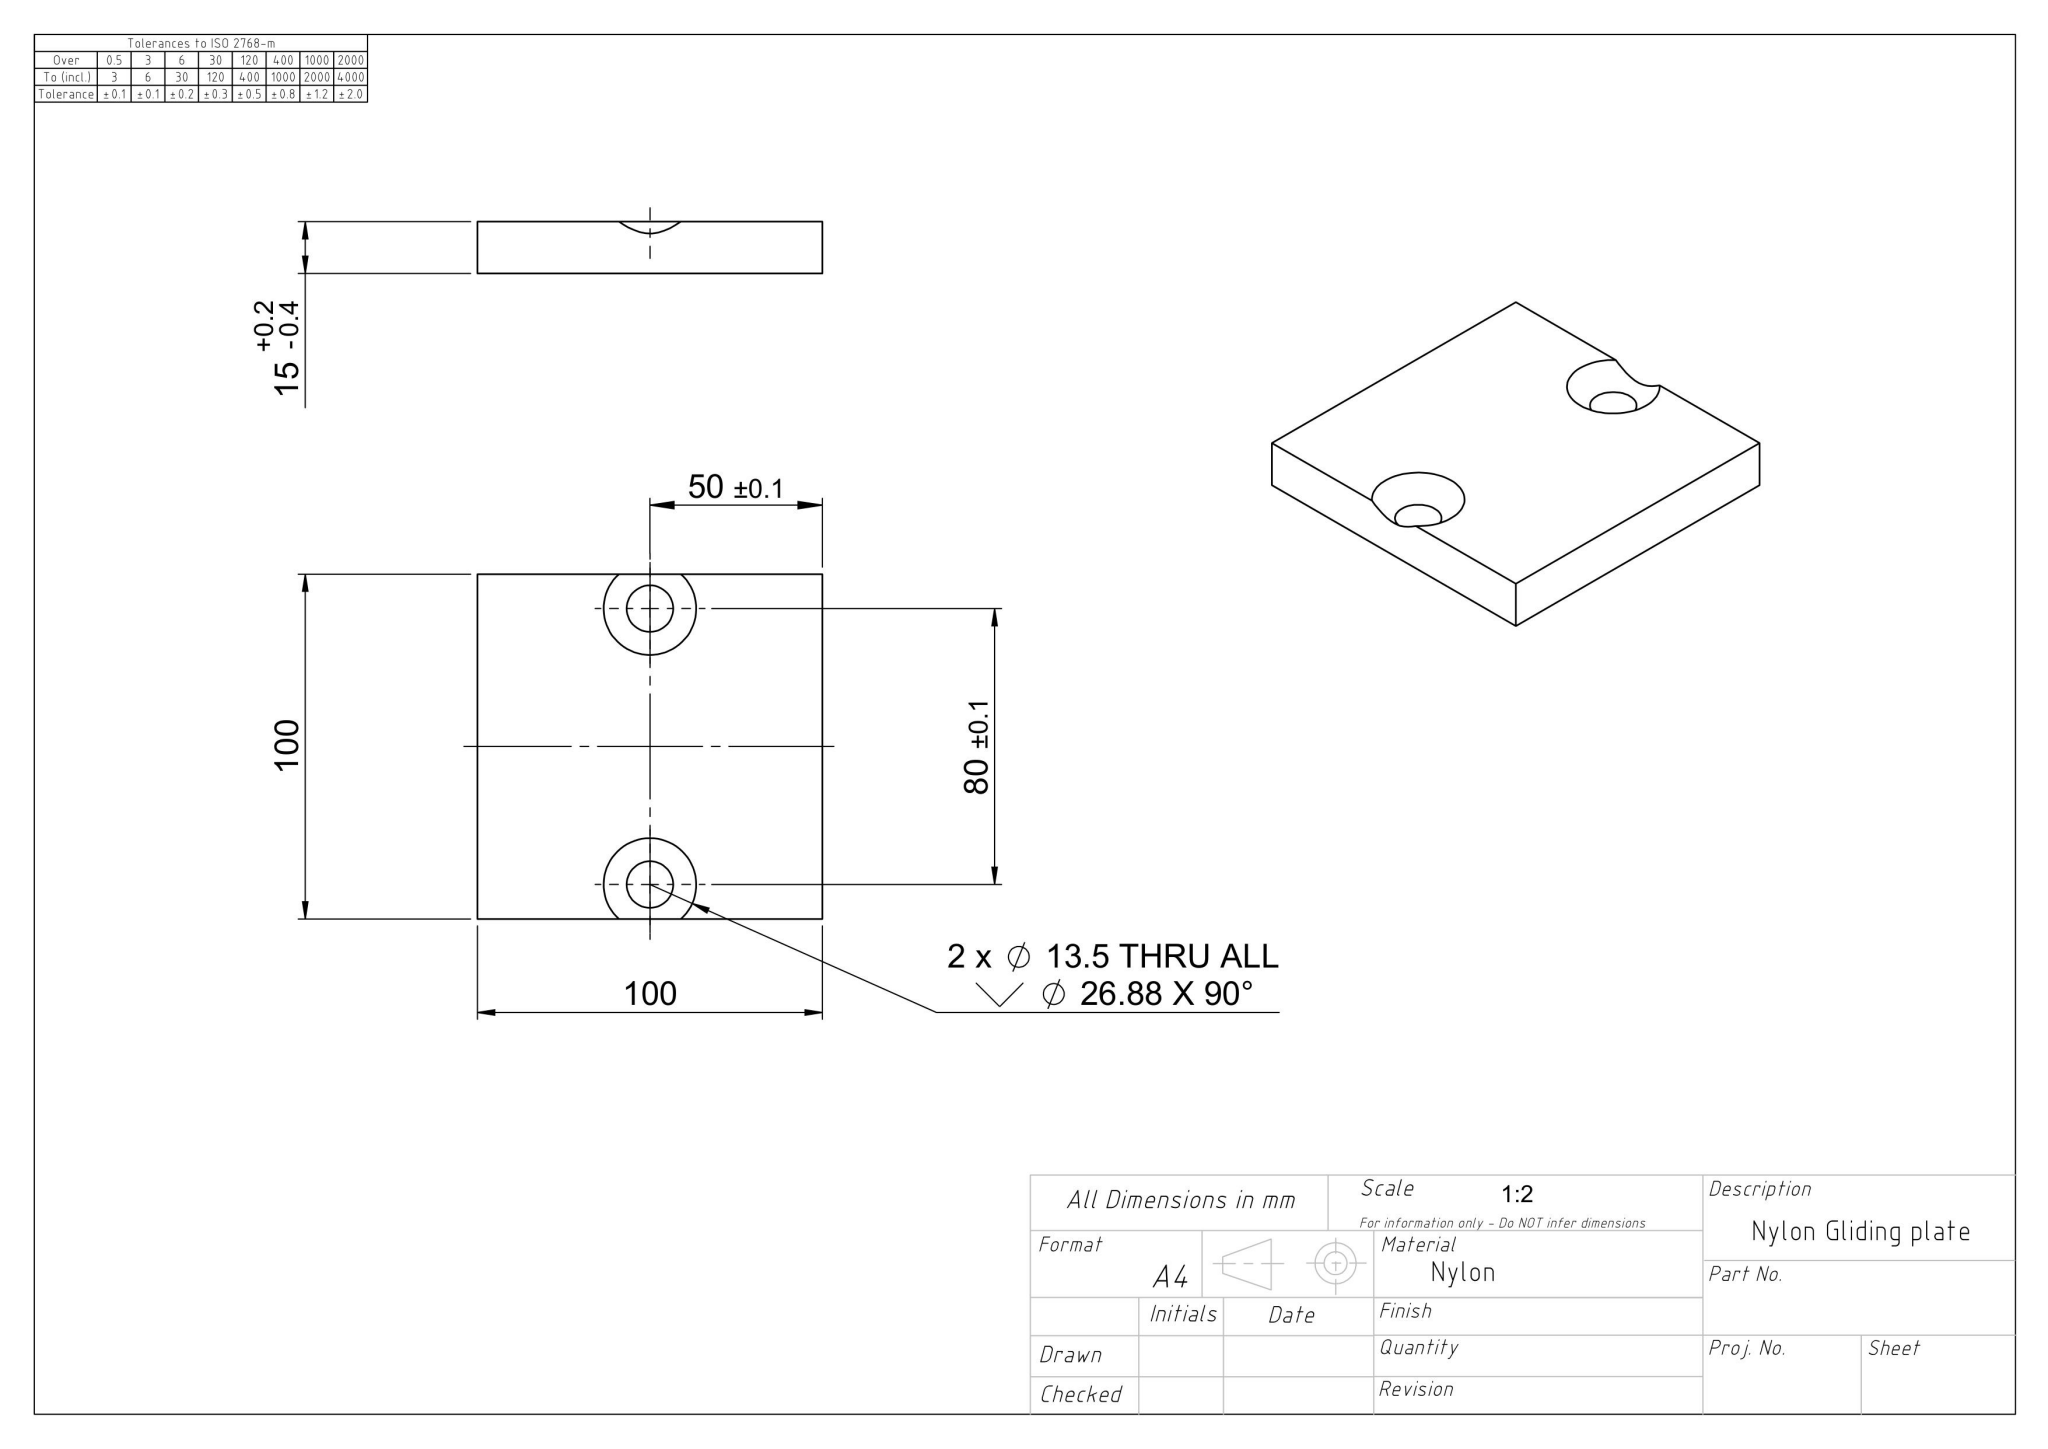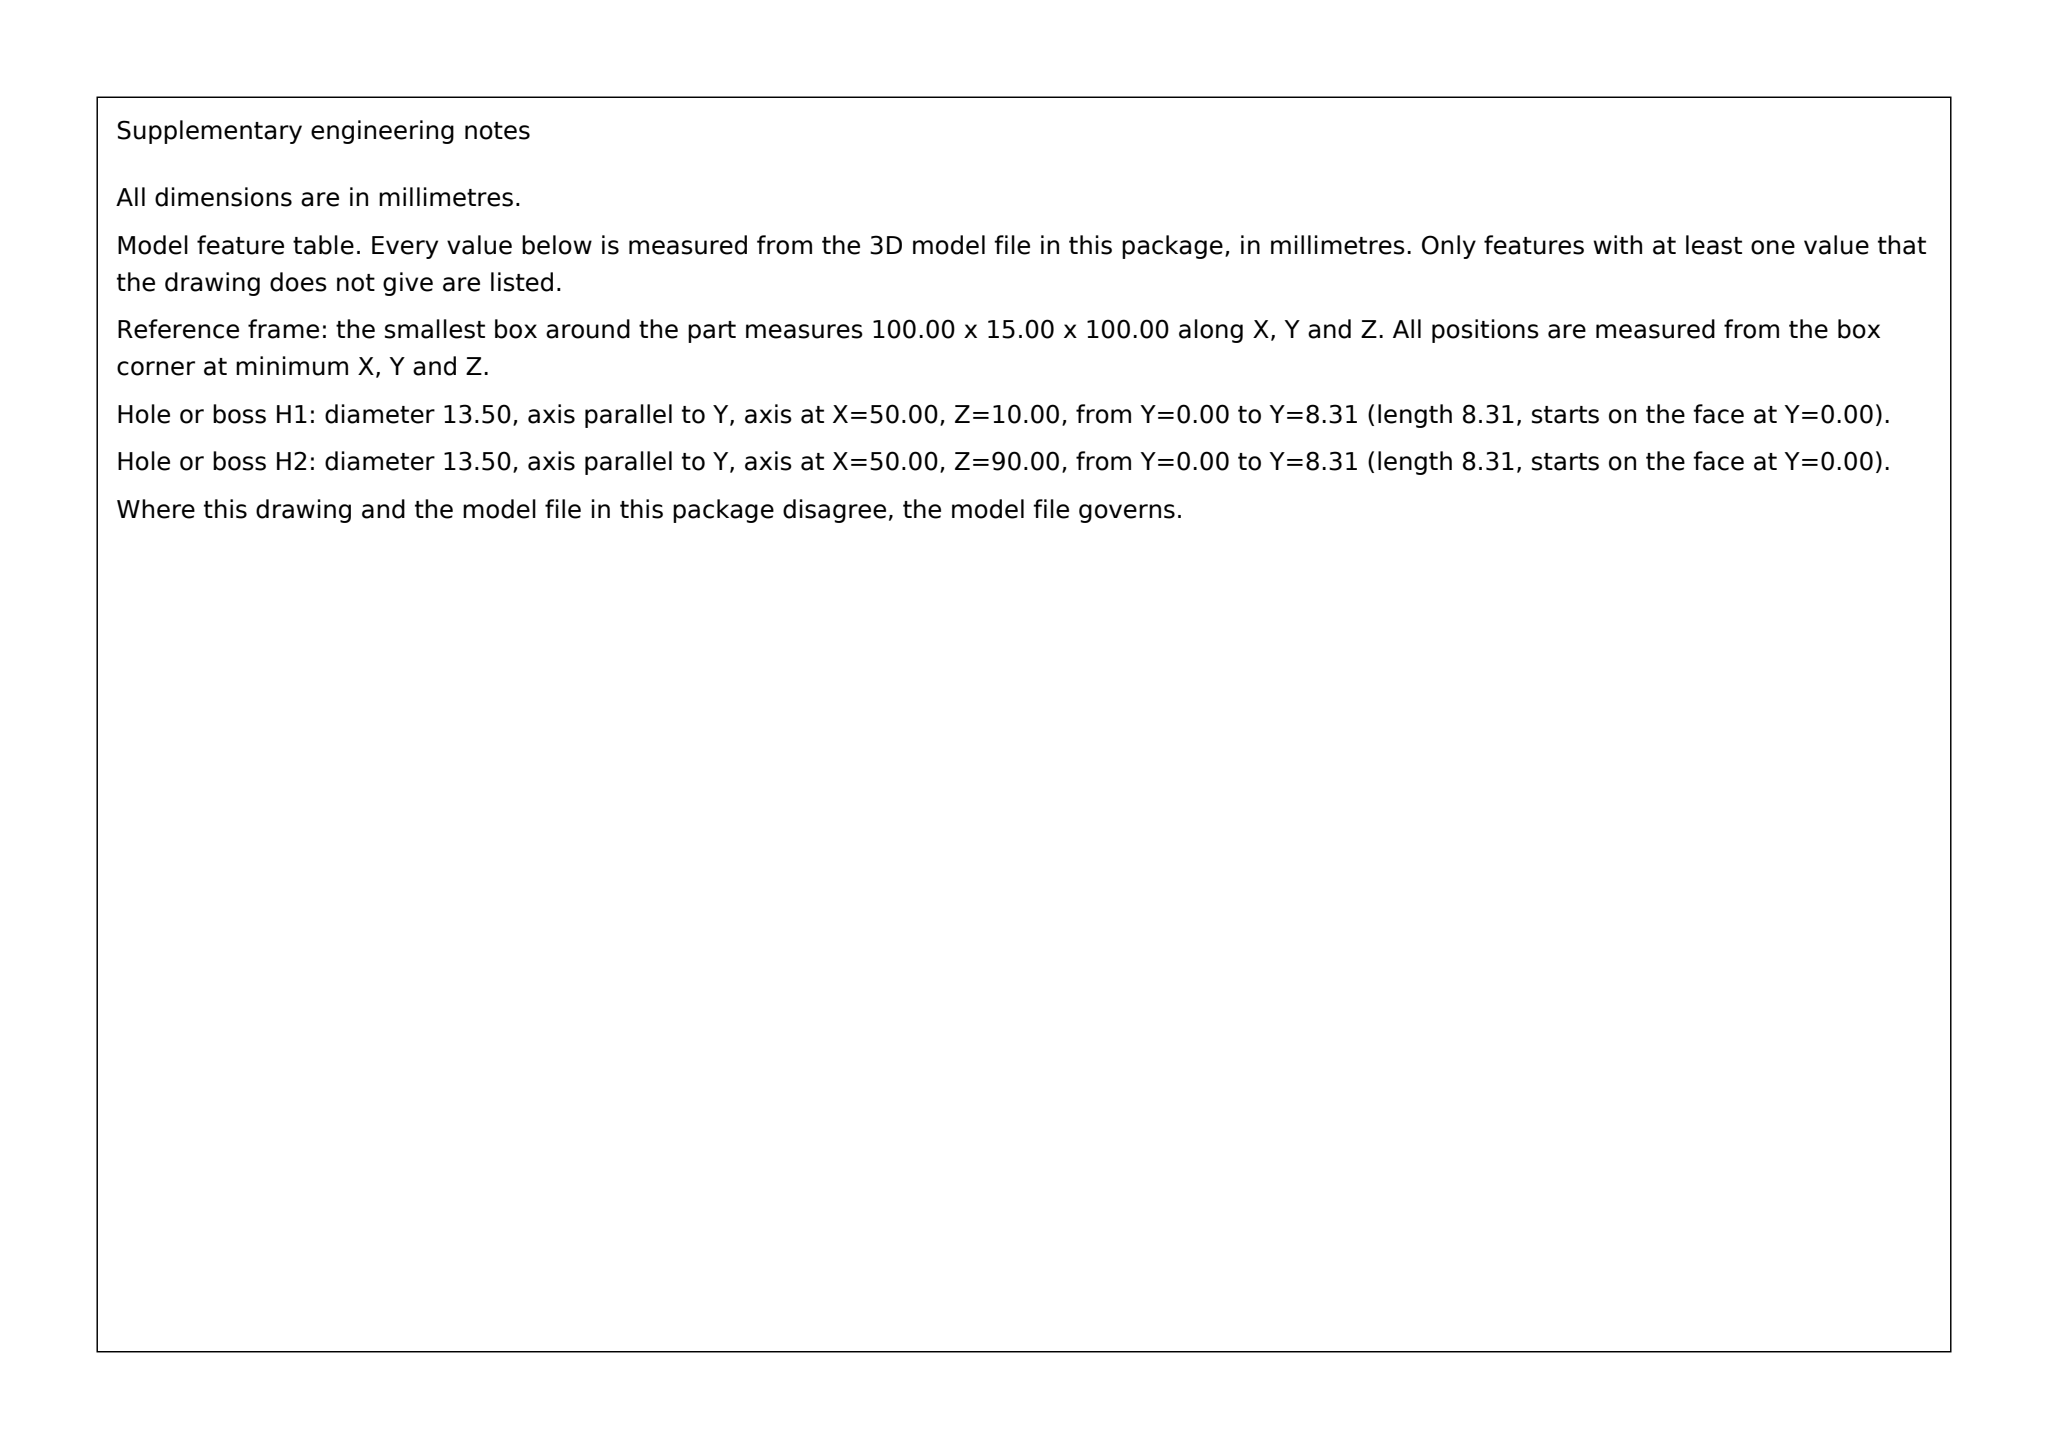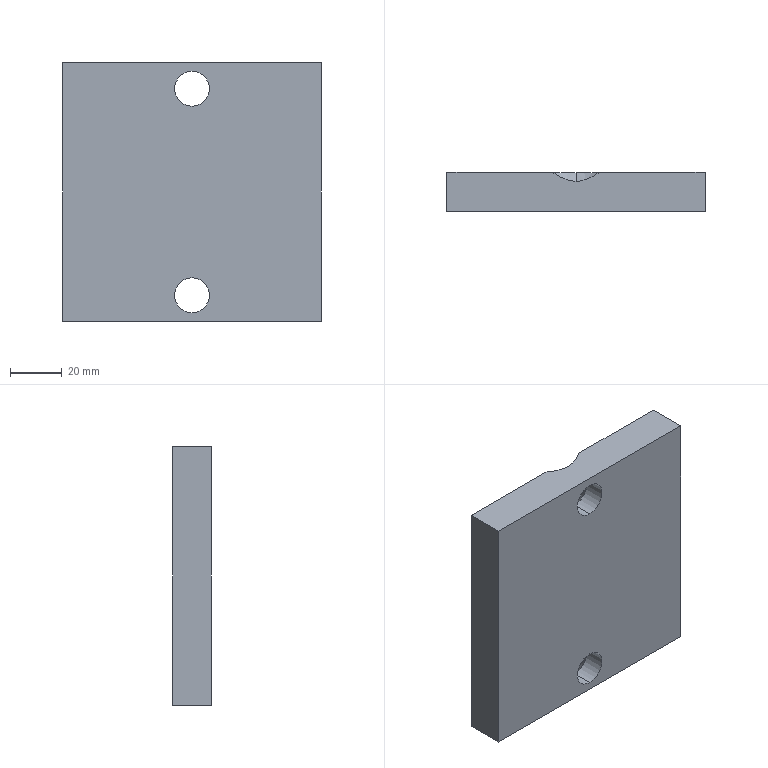Part | SolidWorks | mm | material Nylon | 1 solid | 14 faces | box 100 x 15 x 100 mm | volume 143294 mm3 | plane 6 | cylinder 4 | cone 4 | commonest cylinder face diameters 13.5 x4
build123d program:
from build123d import *

# Parameters (mm, degrees)
SKETCH4_W                                            = 100
SKETCH4_H                                            = 100
BOSS_EXTRUDE3_DEPTH                                  = 15
CSK_FOR_M12_HEX_SOCKET_COUNTERSUNK_CAP_S_D           = 13.5
CSK_FOR_M12_HEX_SOCKET_COUNTERSUNK_CAP_S_CSINK_D     = 26.88
CSK_FOR_M12_HEX_SOCKET_COUNTERSUNK_CAP_S_CSINK_ANGLE = 90


with BuildPart() as part:
    # Sketch4 → Boss-Extrude3 (new body)
    with BuildSketch(Plane(origin=(0, 0, 0), x_dir=(1, 0, 0), z_dir=(0, 1, 0))):
        Rectangle(SKETCH4_W, SKETCH4_H)
    extrude(amount=BOSS_EXTRUDE3_DEPTH)

    # CSK for M12 Hex Socket Countersunk Cap S (through all)
    with Locations(Plane(origin=(0, 15, 0), x_dir=(1, 0, 0), z_dir=(0, 1, 0))):
        with Locations((0, 40), (0, -40)):
            CounterSinkHole(CSK_FOR_M12_HEX_SOCKET_COUNTERSUNK_CAP_S_D / 2, CSK_FOR_M12_HEX_SOCKET_COUNTERSUNK_CAP_S_CSINK_D / 2, counter_sink_angle=CSK_FOR_M12_HEX_SOCKET_COUNTERSUNK_CAP_S_CSINK_ANGLE)


solid = part.part
STEP:
#1=CARTESIAN_POINT('',(0.,0.,-46.75));
#2=VERTEX_POINT('',#1);
#3=CARTESIAN_POINT('',(0.,0.,-33.25));
#4=VERTEX_POINT('',#3);
#5=CARTESIAN_POINT('',(0.,0.,-40.));
#6=DIRECTION('',(0.,1.,0.));
#7=DIRECTION('',(0.,0.,1.));
#8=AXIS2_PLACEMENT_3D('',#5,#6,#7);
#9=CIRCLE('',#8,6.75);
#10=EDGE_CURVE('',#2,#4,#9,.T.);
#11=ORIENTED_EDGE('',*,*,#10,.F.);
#12=CARTESIAN_POINT('',(0.,8.31,-46.75));
#13=VERTEX_POINT('',#12);
#14=CARTESIAN_POINT('',(0.,15.,-46.75));
#15=DIRECTION('',(0.,1.,0.));
#16=VECTOR('',#15,1000.);
#17=LINE('',#14,#16);
#18=EDGE_CURVE('',#2,#13,#17,.T.);
#19=ORIENTED_EDGE('',*,*,#18,.T.);
#20=CARTESIAN_POINT('',(0.,8.31,-33.25));
#21=VERTEX_POINT('',#20);
#22=CARTESIAN_POINT('',(0.,8.31,-40.));
#23=DIRECTION('',(0.,1.,0.));
#24=DIRECTION('',(0.,0.,1.));
#25=AXIS2_PLACEMENT_3D('',#22,#23,#24);
#26=CIRCLE('',#25,6.75);
#27=EDGE_CURVE('',#13,#21,#26,.T.);
#28=ORIENTED_EDGE('',*,*,#27,.T.);
#29=CARTESIAN_POINT('',(0.,15.,-33.25));
#30=DIRECTION('',(0.,1.,0.));
#31=VECTOR('',#30,1000.);
#32=LINE('',#29,#31);
#33=EDGE_CURVE('',#4,#21,#32,.T.);
#34=ORIENTED_EDGE('',*,*,#33,.F.);
#35=EDGE_LOOP('',(#11,#19,#28,#34));
#36=FACE_OUTER_BOUND('',#35,.T.);
#37=CARTESIAN_POINT('',(0.,15.,-40.));
#38=DIRECTION('',(0.,1.,0.));
#39=DIRECTION('',(0.,0.,1.));
#40=AXIS2_PLACEMENT_3D('',#37,#38,#39);
#41=CYLINDRICAL_SURFACE('',#40,6.75);
#42=ADVANCED_FACE('',(#36),#41,.F.);
#43=ORIENTED_EDGE('',*,*,#27,.F.);
#44=CARTESIAN_POINT('',(0.,11.56,-50.));
#45=VERTEX_POINT('',#44);
#46=CARTESIAN_POINT('',(0.,15.,-53.44));
#47=DIRECTION('',(0.,0.7071,-0.7071));
#48=VECTOR('',#47,1000.);
#49=LINE('',#46,#48);
#50=EDGE_CURVE('',#13,#45,#49,.T.);
#51=ORIENTED_EDGE('',*,*,#50,.T.);
#52=CARTESIAN_POINT('',(-8.98,15.,-50.));
#53=VERTEX_POINT('',#52);
#54=CARTESIAN_POINT('',(-8.98,15.,-50.));
#55=CARTESIAN_POINT('',(-8.304,14.548,-50.));
#56=CARTESIAN_POINT('',(-7.611,14.114,-50.));
#57=CARTESIAN_POINT('',(-6.197,13.31,-50.));
#58=CARTESIAN_POINT('',(-5.475,12.941,-50.));
#59=CARTESIAN_POINT('',(-4.357,12.463,-50.));
#60=CARTESIAN_POINT('',(-3.978,12.316,-50.));
#61=CARTESIAN_POINT('',(-3.206,12.055,-50.));
#62=CARTESIAN_POINT('',(-2.81,11.94,-50.));
#63=CARTESIAN_POINT('',(-1.619,11.661,-50.));
#64=CARTESIAN_POINT('',(-0.8152,11.56,-50.));
#65=CARTESIAN_POINT('',(0.,11.56,-50.));
#66=B_SPLINE_CURVE_WITH_KNOTS('',3,(#54,#55,#56,#57,#58,#59,#60,#61,#62,#63,#64,#65),.UNSPECIFIED.,.F.,.F.,(4,2,2,2,2,4),(0.01358,0.01601,0.01844,0.01966,0.02087,0.0233),.UNSPECIFIED.);
#67=EDGE_CURVE('',#53,#45,#66,.T.);
#68=ORIENTED_EDGE('',*,*,#67,.F.);
#69=CARTESIAN_POINT('',(0.,15.,-26.56));
#70=VERTEX_POINT('',#69);
#71=CARTESIAN_POINT('',(0.,15.,-40.));
#72=DIRECTION('',(0.,1.,0.));
#73=DIRECTION('',(0.,0.,1.));
#74=AXIS2_PLACEMENT_3D('',#71,#72,#73);
#75=CIRCLE('',#74,13.44);
#76=EDGE_CURVE('',#53,#70,#75,.T.);
#77=ORIENTED_EDGE('',*,*,#76,.T.);
#78=CARTESIAN_POINT('',(0.,15.,-26.56));
#79=DIRECTION('',(0.,0.7071,0.7071));
#80=VECTOR('',#79,1000.);
#81=LINE('',#78,#80);
#82=EDGE_CURVE('',#21,#70,#81,.T.);
#83=ORIENTED_EDGE('',*,*,#82,.F.);
#84=EDGE_LOOP('',(#43,#51,#68,#77,#83));
#85=FACE_OUTER_BOUND('',#84,.T.);
#86=CARTESIAN_POINT('',(0.,15.,-40.));
#87=DIRECTION('',(0.,1.,0.));
#88=DIRECTION('',(0.,0.,1.));
#89=AXIS2_PLACEMENT_3D('',#86,#87,#88);
#90=CONICAL_SURFACE('',#89,13.44,0.7854);
#91=ADVANCED_FACE('',(#85),#90,.F.);
#92=CARTESIAN_POINT('',(0.,0.,33.25));
#93=VERTEX_POINT('',#92);
#94=CARTESIAN_POINT('',(0.,0.,46.75));
#95=VERTEX_POINT('',#94);
#96=CARTESIAN_POINT('',(0.,0.,40.));
#97=DIRECTION('',(0.,1.,0.));
#98=DIRECTION('',(0.,0.,1.));
#99=AXIS2_PLACEMENT_3D('',#96,#97,#98);
#100=CIRCLE('',#99,6.75);
#101=EDGE_CURVE('',#93,#95,#100,.T.);
#102=ORIENTED_EDGE('',*,*,#101,.F.);
#103=CARTESIAN_POINT('',(0.,8.31,33.25));
#104=VERTEX_POINT('',#103);
#105=CARTESIAN_POINT('',(0.,15.,33.25));
#106=DIRECTION('',(0.,1.,0.));
#107=VECTOR('',#106,1000.);
#108=LINE('',#105,#107);
#109=EDGE_CURVE('',#93,#104,#108,.T.);
#110=ORIENTED_EDGE('',*,*,#109,.T.);
#111=CARTESIAN_POINT('',(0.,8.31,46.75));
#112=VERTEX_POINT('',#111);
#113=CARTESIAN_POINT('',(0.,8.31,40.));
#114=DIRECTION('',(0.,1.,0.));
#115=DIRECTION('',(0.,0.,1.));
#116=AXIS2_PLACEMENT_3D('',#113,#114,#115);
#117=CIRCLE('',#116,6.75);
#118=EDGE_CURVE('',#104,#112,#117,.T.);
#119=ORIENTED_EDGE('',*,*,#118,.T.);
#120=CARTESIAN_POINT('',(0.,15.,46.75));
#121=DIRECTION('',(0.,1.,0.));
#122=VECTOR('',#121,1000.);
#123=LINE('',#120,#122);
#124=EDGE_CURVE('',#95,#112,#123,.T.);
#125=ORIENTED_EDGE('',*,*,#124,.F.);
#126=EDGE_LOOP('',(#102,#110,#119,#125));
#127=FACE_OUTER_BOUND('',#126,.T.);
#128=CARTESIAN_POINT('',(0.,15.,40.));
#129=DIRECTION('',(0.,1.,0.));
#130=DIRECTION('',(0.,0.,1.));
#131=AXIS2_PLACEMENT_3D('',#128,#129,#130);
#132=CYLINDRICAL_SURFACE('',#131,6.75);
#133=ADVANCED_FACE('',(#127),#132,.F.);
#134=ORIENTED_EDGE('',*,*,#118,.F.);
#135=CARTESIAN_POINT('',(0.,15.,26.56));
#136=VERTEX_POINT('',#135);
#137=CARTESIAN_POINT('',(0.,15.,26.56));
#138=DIRECTION('',(0.,0.7071,-0.7071));
#139=VECTOR('',#138,1000.);
#140=LINE('',#137,#139);
#141=EDGE_CURVE('',#104,#136,#140,.T.);
#142=ORIENTED_EDGE('',*,*,#141,.T.);
#143=CARTESIAN_POINT('',(-8.98,15.,50.));
#144=VERTEX_POINT('',#143);
#145=CARTESIAN_POINT('',(0.,15.,40.));
#146=DIRECTION('',(0.,1.,0.));
#147=DIRECTION('',(0.,0.,1.));
#148=AXIS2_PLACEMENT_3D('',#145,#146,#147);
#149=CIRCLE('',#148,13.44);
#150=EDGE_CURVE('',#136,#144,#149,.T.);
#151=ORIENTED_EDGE('',*,*,#150,.T.);
#152=CARTESIAN_POINT('',(0.,11.56,50.));
#153=VERTEX_POINT('',#152);
#154=CARTESIAN_POINT('',(0.,11.56,50.));
#155=CARTESIAN_POINT('',(-0.8152,11.56,50.));
#156=CARTESIAN_POINT('',(-1.619,11.661,50.));
#157=CARTESIAN_POINT('',(-2.81,11.94,50.));
#158=CARTESIAN_POINT('',(-3.206,12.055,50.));
#159=CARTESIAN_POINT('',(-3.978,12.316,50.));
#160=CARTESIAN_POINT('',(-4.357,12.463,50.));
#161=CARTESIAN_POINT('',(-5.475,12.941,50.));
#162=CARTESIAN_POINT('',(-6.197,13.31,50.));
#163=CARTESIAN_POINT('',(-7.611,14.114,50.));
#164=CARTESIAN_POINT('',(-8.304,14.548,50.));
#165=CARTESIAN_POINT('',(-8.98,15.,50.));
#166=B_SPLINE_CURVE_WITH_KNOTS('',3,(#154,#155,#156,#157,#158,#159,#160,#161,#162,#163,#164,#165),.UNSPECIFIED.,.F.,.F.,(4,2,2,2,2,4),(0.05657,0.059,0.06021,0.06142,0.06384,0.06626),.UNSPECIFIED.);
#167=EDGE_CURVE('',#153,#144,#166,.T.);
#168=ORIENTED_EDGE('',*,*,#167,.F.);
#169=CARTESIAN_POINT('',(0.,15.,53.44));
#170=DIRECTION('',(0.,0.7071,0.7071));
#171=VECTOR('',#170,1000.);
#172=LINE('',#169,#171);
#173=EDGE_CURVE('',#112,#153,#172,.T.);
#174=ORIENTED_EDGE('',*,*,#173,.F.);
#175=EDGE_LOOP('',(#134,#142,#151,#168,#174));
#176=FACE_OUTER_BOUND('',#175,.T.);
#177=CARTESIAN_POINT('',(0.,15.,40.));
#178=DIRECTION('',(0.,1.,0.));
#179=DIRECTION('',(0.,0.,1.));
#180=AXIS2_PLACEMENT_3D('',#177,#178,#179);
#181=CONICAL_SURFACE('',#180,13.44,0.7854);
#182=ADVANCED_FACE('',(#176),#181,.F.);
#183=CARTESIAN_POINT('',(50.,0.,50.));
#184=VERTEX_POINT('',#183);
#185=CARTESIAN_POINT('',(50.,0.,-50.));
#186=VERTEX_POINT('',#185);
#187=CARTESIAN_POINT('',(50.,0.,-50.));
#188=DIRECTION('',(-0.,0.,-1.));
#189=VECTOR('',#188,1000.);
#190=LINE('',#187,#189);
#191=EDGE_CURVE('',#184,#186,#190,.T.);
#192=ORIENTED_EDGE('',*,*,#191,.T.);
#193=CARTESIAN_POINT('',(50.,15.,-50.));
#194=VERTEX_POINT('',#193);
#195=CARTESIAN_POINT('',(50.,15.,-50.));
#196=DIRECTION('',(0.,-1.,0.));
#197=VECTOR('',#196,1000.);
#198=LINE('',#195,#197);
#199=EDGE_CURVE('',#194,#186,#198,.T.);
#200=ORIENTED_EDGE('',*,*,#199,.F.);
#201=CARTESIAN_POINT('',(50.,15.,50.));
#202=VERTEX_POINT('',#201);
#203=CARTESIAN_POINT('',(50.,15.,-50.));
#204=DIRECTION('',(-0.,0.,-1.));
#205=VECTOR('',#204,1000.);
#206=LINE('',#203,#205);
#207=EDGE_CURVE('',#202,#194,#206,.T.);
#208=ORIENTED_EDGE('',*,*,#207,.F.);
#209=CARTESIAN_POINT('',(50.,15.,50.));
#210=DIRECTION('',(0.,-1.,0.));
#211=VECTOR('',#210,1000.);
#212=LINE('',#209,#211);
#213=EDGE_CURVE('',#202,#184,#212,.T.);
#214=ORIENTED_EDGE('',*,*,#213,.T.);
#215=EDGE_LOOP('',(#192,#200,#208,#214));
#216=FACE_OUTER_BOUND('',#215,.T.);
#217=CARTESIAN_POINT('',(50.,15.,-50.));
#218=DIRECTION('',(-1.,0.,0.));
#219=DIRECTION('',(0.,0.,1.));
#220=AXIS2_PLACEMENT_3D('',#217,#218,#219);
#221=PLANE('',#220);
#222=ADVANCED_FACE('',(#216),#221,.F.);
#223=CARTESIAN_POINT('',(-50.,15.,-50.));
#224=VERTEX_POINT('',#223);
#225=CARTESIAN_POINT('',(-50.,15.,-50.));
#226=DIRECTION('',(-1.,0.,0.));
#227=VECTOR('',#226,1000.);
#228=LINE('',#225,#227);
#229=EDGE_CURVE('',#53,#224,#228,.T.);
#230=ORIENTED_EDGE('',*,*,#229,.F.);
#231=ORIENTED_EDGE('',*,*,#67,.T.);
#232=CARTESIAN_POINT('',(8.98,15.,-50.));
#233=VERTEX_POINT('',#232);
#234=CARTESIAN_POINT('',(0.,11.56,-50.));
#235=CARTESIAN_POINT('',(0.4083,11.56,-50.));
#236=CARTESIAN_POINT('',(0.8216,11.586,-50.));
#237=CARTESIAN_POINT('',(1.633,11.685,-50.));
#238=CARTESIAN_POINT('',(2.034,11.757,-50.));
#239=CARTESIAN_POINT('',(2.826,11.944,-50.));
#240=CARTESIAN_POINT('',(3.217,12.058,-50.));
#241=CARTESIAN_POINT('',(3.991,12.321,-50.));
#242=CARTESIAN_POINT('',(4.375,12.47,-50.));
#243=CARTESIAN_POINT('',(5.5,12.952,-50.));
#244=CARTESIAN_POINT('',(6.22,13.322,-50.));
#245=CARTESIAN_POINT('',(7.624,14.122,-50.));
#246=CARTESIAN_POINT('',(8.308,14.551,-50.));
#247=CARTESIAN_POINT('',(8.98,15.,-50.));
#248=B_SPLINE_CURVE_WITH_KNOTS('',3,(#234,#235,#236,#237,#238,#239,#240,#241,#242,#243,#244,#245,#246,#247),.UNSPECIFIED.,.F.,.F.,(4,2,2,2,2,2,4),(0.0233,0.02452,0.02574,0.02696,0.02818,0.03061,0.03305),.UNSPECIFIED.);
#249=EDGE_CURVE('',#45,#233,#248,.T.);
#250=ORIENTED_EDGE('',*,*,#249,.T.);
#251=CARTESIAN_POINT('',(-50.,15.,-50.));
#252=DIRECTION('',(-1.,0.,0.));
#253=VECTOR('',#252,1000.);
#254=LINE('',#251,#253);
#255=EDGE_CURVE('',#194,#233,#254,.T.);
#256=ORIENTED_EDGE('',*,*,#255,.F.);
#257=ORIENTED_EDGE('',*,*,#199,.T.);
#258=CARTESIAN_POINT('',(-50.,0.,-50.));
#259=VERTEX_POINT('',#258);
#260=CARTESIAN_POINT('',(-50.,0.,-50.));
#261=DIRECTION('',(-1.,0.,0.));
#262=VECTOR('',#261,1000.);
#263=LINE('',#260,#262);
#264=EDGE_CURVE('',#186,#259,#263,.T.);
#265=ORIENTED_EDGE('',*,*,#264,.T.);
#266=CARTESIAN_POINT('',(-50.,15.,-50.));
#267=DIRECTION('',(0.,-1.,0.));
#268=VECTOR('',#267,1000.);
#269=LINE('',#266,#268);
#270=EDGE_CURVE('',#224,#259,#269,.T.);
#271=ORIENTED_EDGE('',*,*,#270,.F.);
#272=EDGE_LOOP('',(#230,#231,#250,#256,#257,#265,#271));
#273=FACE_OUTER_BOUND('',#272,.T.);
#274=CARTESIAN_POINT('',(-50.,15.,-50.));
#275=DIRECTION('',(0.,0.,1.));
#276=DIRECTION('',(1.,0.,0.));
#277=AXIS2_PLACEMENT_3D('',#274,#275,#276);
#278=PLANE('',#277);
#279=ADVANCED_FACE('',(#273),#278,.F.);
#280=CARTESIAN_POINT('',(-50.,0.,50.));
#281=VERTEX_POINT('',#280);
#282=CARTESIAN_POINT('',(-50.,0.,-50.));
#283=DIRECTION('',(0.,0.,1.));
#284=VECTOR('',#283,1000.);
#285=LINE('',#282,#284);
#286=EDGE_CURVE('',#259,#281,#285,.T.);
#287=ORIENTED_EDGE('',*,*,#286,.T.);
#288=CARTESIAN_POINT('',(-50.,15.,50.));
#289=VERTEX_POINT('',#288);
#290=CARTESIAN_POINT('',(-50.,15.,50.));
#291=DIRECTION('',(0.,-1.,0.));
#292=VECTOR('',#291,1000.);
#293=LINE('',#290,#292);
#294=EDGE_CURVE('',#289,#281,#293,.T.);
#295=ORIENTED_EDGE('',*,*,#294,.F.);
#296=CARTESIAN_POINT('',(-50.,15.,-50.));
#297=DIRECTION('',(0.,0.,1.));
#298=VECTOR('',#297,1000.);
#299=LINE('',#296,#298);
#300=EDGE_CURVE('',#224,#289,#299,.T.);
#301=ORIENTED_EDGE('',*,*,#300,.F.);
#302=ORIENTED_EDGE('',*,*,#270,.T.);
#303=EDGE_LOOP('',(#287,#295,#301,#302));
#304=FACE_OUTER_BOUND('',#303,.T.);
#305=CARTESIAN_POINT('',(-50.,15.,-50.));
#306=DIRECTION('',(1.,0.,0.));
#307=DIRECTION('',(0.,0.,-1.));
#308=AXIS2_PLACEMENT_3D('',#305,#306,#307);
#309=PLANE('',#308);
#310=ADVANCED_FACE('',(#304),#309,.F.);
#311=CARTESIAN_POINT('',(8.98,15.,50.));
#312=VERTEX_POINT('',#311);
#313=CARTESIAN_POINT('',(-50.,15.,50.));
#314=DIRECTION('',(1.,0.,0.));
#315=VECTOR('',#314,1000.);
#316=LINE('',#313,#315);
#317=EDGE_CURVE('',#312,#202,#316,.T.);
#318=ORIENTED_EDGE('',*,*,#317,.F.);
#319=CARTESIAN_POINT('',(8.98,15.,50.));
#320=CARTESIAN_POINT('',(8.308,14.551,50.));
#321=CARTESIAN_POINT('',(7.624,14.122,50.));
#322=CARTESIAN_POINT('',(6.22,13.322,50.));
#323=CARTESIAN_POINT('',(5.5,12.952,50.));
#324=CARTESIAN_POINT('',(4.375,12.47,50.));
#325=CARTESIAN_POINT('',(3.991,12.321,50.));
#326=CARTESIAN_POINT('',(3.217,12.058,50.));
#327=CARTESIAN_POINT('',(2.826,11.944,50.));
#328=CARTESIAN_POINT('',(2.034,11.757,50.));
#329=CARTESIAN_POINT('',(1.633,11.685,50.));
#330=CARTESIAN_POINT('',(0.8216,11.586,50.));
#331=CARTESIAN_POINT('',(0.4083,11.56,50.));
#332=CARTESIAN_POINT('',(0.,11.56,50.));
#333=B_SPLINE_CURVE_WITH_KNOTS('',3,(#319,#320,#321,#322,#323,#324,#325,#326,#327,#328,#329,#330,#331,#332),.UNSPECIFIED.,.F.,.F.,(4,2,2,2,2,2,4),(0.04686,0.04929,0.05172,0.05293,0.05415,0.05536,0.05657),.UNSPECIFIED.);
#334=EDGE_CURVE('',#312,#153,#333,.T.);
#335=ORIENTED_EDGE('',*,*,#334,.T.);
#336=ORIENTED_EDGE('',*,*,#167,.T.);
#337=CARTESIAN_POINT('',(-50.,15.,50.));
#338=DIRECTION('',(1.,0.,0.));
#339=VECTOR('',#338,1000.);
#340=LINE('',#337,#339);
#341=EDGE_CURVE('',#289,#144,#340,.T.);
#342=ORIENTED_EDGE('',*,*,#341,.F.);
#343=ORIENTED_EDGE('',*,*,#294,.T.);
#344=CARTESIAN_POINT('',(-50.,0.,50.));
#345=DIRECTION('',(1.,0.,0.));
#346=VECTOR('',#345,1000.);
#347=LINE('',#344,#346);
#348=EDGE_CURVE('',#281,#184,#347,.T.);
#349=ORIENTED_EDGE('',*,*,#348,.T.);
#350=ORIENTED_EDGE('',*,*,#213,.F.);
#351=EDGE_LOOP('',(#318,#335,#336,#342,#343,#349,#350));
#352=FACE_OUTER_BOUND('',#351,.T.);
#353=CARTESIAN_POINT('',(-50.,15.,50.));
#354=DIRECTION('',(0.,0.,-1.));
#355=DIRECTION('',(-1.,0.,0.));
#356=AXIS2_PLACEMENT_3D('',#353,#354,#355);
#357=PLANE('',#356);
#358=ADVANCED_FACE('',(#352),#357,.F.);
#359=ORIENTED_EDGE('',*,*,#76,.F.);
#360=ORIENTED_EDGE('',*,*,#229,.T.);
#361=ORIENTED_EDGE('',*,*,#300,.T.);
#362=ORIENTED_EDGE('',*,*,#341,.T.);
#363=ORIENTED_EDGE('',*,*,#150,.F.);
#364=CARTESIAN_POINT('',(0.,15.,40.));
#365=DIRECTION('',(0.,1.,0.));
#366=DIRECTION('',(0.,0.,1.));
#367=AXIS2_PLACEMENT_3D('',#364,#365,#366);
#368=CIRCLE('',#367,13.44);
#369=EDGE_CURVE('',#312,#136,#368,.T.);
#370=ORIENTED_EDGE('',*,*,#369,.F.);
#371=ORIENTED_EDGE('',*,*,#317,.T.);
#372=ORIENTED_EDGE('',*,*,#207,.T.);
#373=ORIENTED_EDGE('',*,*,#255,.T.);
#374=CARTESIAN_POINT('',(0.,15.,-40.));
#375=DIRECTION('',(0.,1.,0.));
#376=DIRECTION('',(0.,0.,1.));
#377=AXIS2_PLACEMENT_3D('',#374,#375,#376);
#378=CIRCLE('',#377,13.44);
#379=EDGE_CURVE('',#70,#233,#378,.T.);
#380=ORIENTED_EDGE('',*,*,#379,.F.);
#381=EDGE_LOOP('',(#359,#360,#361,#362,#363,#370,#371,#372,#373,#380));
#382=FACE_OUTER_BOUND('',#381,.T.);
#383=CARTESIAN_POINT('',(0.,15.,0.));
#384=DIRECTION('',(0.,1.,0.));
#385=DIRECTION('',(0.,0.,1.));
#386=AXIS2_PLACEMENT_3D('',#383,#384,#385);
#387=PLANE('',#386);
#388=ADVANCED_FACE('',(#382),#387,.T.);
#389=CARTESIAN_POINT('',(0.,0.,-40.));
#390=DIRECTION('',(0.,1.,0.));
#391=DIRECTION('',(0.,0.,1.));
#392=AXIS2_PLACEMENT_3D('',#389,#390,#391);
#393=CIRCLE('',#392,6.75);
#394=EDGE_CURVE('',#4,#2,#393,.T.);
#395=ORIENTED_EDGE('',*,*,#394,.T.);
#396=ORIENTED_EDGE('',*,*,#10,.T.);
#397=EDGE_LOOP('',(#395,#396));
#398=FACE_BOUND('',#397,.T.);
#399=CARTESIAN_POINT('',(0.,0.,40.));
#400=DIRECTION('',(0.,1.,0.));
#401=DIRECTION('',(0.,0.,1.));
#402=AXIS2_PLACEMENT_3D('',#399,#400,#401);
#403=CIRCLE('',#402,6.75);
#404=EDGE_CURVE('',#95,#93,#403,.T.);
#405=ORIENTED_EDGE('',*,*,#404,.T.);
#406=ORIENTED_EDGE('',*,*,#101,.T.);
#407=EDGE_LOOP('',(#405,#406));
#408=FACE_BOUND('',#407,.T.);
#409=ORIENTED_EDGE('',*,*,#191,.F.);
#410=ORIENTED_EDGE('',*,*,#348,.F.);
#411=ORIENTED_EDGE('',*,*,#286,.F.);
#412=ORIENTED_EDGE('',*,*,#264,.F.);
#413=EDGE_LOOP('',(#409,#410,#411,#412));
#414=FACE_OUTER_BOUND('',#413,.T.);
#415=CARTESIAN_POINT('',(0.,0.,0.));
#416=DIRECTION('',(0.,1.,0.));
#417=DIRECTION('',(0.,0.,1.));
#418=AXIS2_PLACEMENT_3D('',#415,#416,#417);
#419=PLANE('',#418);
#420=ADVANCED_FACE('',(#398,#408,#414),#419,.F.);
#421=ORIENTED_EDGE('',*,*,#141,.F.);
#422=CARTESIAN_POINT('',(0.,8.31,40.));
#423=DIRECTION('',(0.,1.,0.));
#424=DIRECTION('',(0.,0.,1.));
#425=AXIS2_PLACEMENT_3D('',#422,#423,#424);
#426=CIRCLE('',#425,6.75);
#427=EDGE_CURVE('',#112,#104,#426,.T.);
#428=ORIENTED_EDGE('',*,*,#427,.F.);
#429=ORIENTED_EDGE('',*,*,#173,.T.);
#430=ORIENTED_EDGE('',*,*,#334,.F.);
#431=ORIENTED_EDGE('',*,*,#369,.T.);
#432=EDGE_LOOP('',(#421,#428,#429,#430,#431));
#433=FACE_OUTER_BOUND('',#432,.T.);
#434=CARTESIAN_POINT('',(0.,15.,40.));
#435=DIRECTION('',(0.,1.,0.));
#436=DIRECTION('',(0.,0.,1.));
#437=AXIS2_PLACEMENT_3D('',#434,#435,#436);
#438=CONICAL_SURFACE('',#437,13.44,0.7854);
#439=ADVANCED_FACE('',(#433),#438,.F.);
#440=ORIENTED_EDGE('',*,*,#109,.F.);
#441=ORIENTED_EDGE('',*,*,#404,.F.);
#442=ORIENTED_EDGE('',*,*,#124,.T.);
#443=ORIENTED_EDGE('',*,*,#427,.T.);
#444=EDGE_LOOP('',(#440,#441,#442,#443));
#445=FACE_OUTER_BOUND('',#444,.T.);
#446=CARTESIAN_POINT('',(0.,15.,40.));
#447=DIRECTION('',(0.,1.,0.));
#448=DIRECTION('',(0.,0.,1.));
#449=AXIS2_PLACEMENT_3D('',#446,#447,#448);
#450=CYLINDRICAL_SURFACE('',#449,6.75);
#451=ADVANCED_FACE('',(#445),#450,.F.);
#452=ORIENTED_EDGE('',*,*,#50,.F.);
#453=CARTESIAN_POINT('',(0.,8.31,-40.));
#454=DIRECTION('',(0.,1.,0.));
#455=DIRECTION('',(0.,0.,1.));
#456=AXIS2_PLACEMENT_3D('',#453,#454,#455);
#457=CIRCLE('',#456,6.75);
#458=EDGE_CURVE('',#21,#13,#457,.T.);
#459=ORIENTED_EDGE('',*,*,#458,.F.);
#460=ORIENTED_EDGE('',*,*,#82,.T.);
#461=ORIENTED_EDGE('',*,*,#379,.T.);
#462=ORIENTED_EDGE('',*,*,#249,.F.);
#463=EDGE_LOOP('',(#452,#459,#460,#461,#462));
#464=FACE_OUTER_BOUND('',#463,.T.);
#465=CARTESIAN_POINT('',(0.,15.,-40.));
#466=DIRECTION('',(0.,1.,0.));
#467=DIRECTION('',(0.,0.,1.));
#468=AXIS2_PLACEMENT_3D('',#465,#466,#467);
#469=CONICAL_SURFACE('',#468,13.44,0.7854);
#470=ADVANCED_FACE('',(#464),#469,.F.);
#471=ORIENTED_EDGE('',*,*,#18,.F.);
#472=ORIENTED_EDGE('',*,*,#394,.F.);
#473=ORIENTED_EDGE('',*,*,#33,.T.);
#474=ORIENTED_EDGE('',*,*,#458,.T.);
#475=EDGE_LOOP('',(#471,#472,#473,#474));
#476=FACE_OUTER_BOUND('',#475,.T.);
#477=CARTESIAN_POINT('',(0.,15.,-40.));
#478=DIRECTION('',(0.,1.,0.));
#479=DIRECTION('',(0.,0.,1.));
#480=AXIS2_PLACEMENT_3D('',#477,#478,#479);
#481=CYLINDRICAL_SURFACE('',#480,6.75);
#482=ADVANCED_FACE('',(#476),#481,.F.);
#483=CLOSED_SHELL('',(#42,#91,#133,#182,#222,#279,#310,#358,#388,#420,#439,#451,#470,#482));
#484=MANIFOLD_SOLID_BREP('',#483);
#485=CARTESIAN_POINT('',(0.,0.,0.));
#486=DIRECTION('',(0.,0.,1.));
#487=DIRECTION('',(1.,0.,0.));
#488=AXIS2_PLACEMENT_3D('',#485,#486,#487);
#489=(LENGTH_UNIT()NAMED_UNIT(*)SI_UNIT(.MILLI.,.METRE.));
#490=UNCERTAINTY_MEASURE_WITH_UNIT(LENGTH_MEASURE(0.00001),#489,'','');
#491=(NAMED_UNIT(*)PLANE_ANGLE_UNIT()SI_UNIT($,.RADIAN.));
#492=(NAMED_UNIT(*)SI_UNIT($,.STERADIAN.)SOLID_ANGLE_UNIT());
#493=(GEOMETRIC_REPRESENTATION_CONTEXT(3)GLOBAL_UNCERTAINTY_ASSIGNED_CONTEXT((#490))GLOBAL_UNIT_ASSIGNED_CONTEXT((#489,#491,#492))REPRESENTATION_CONTEXT('',''));
#494=ADVANCED_BREP_SHAPE_REPRESENTATION('',(#484,#488),#493);